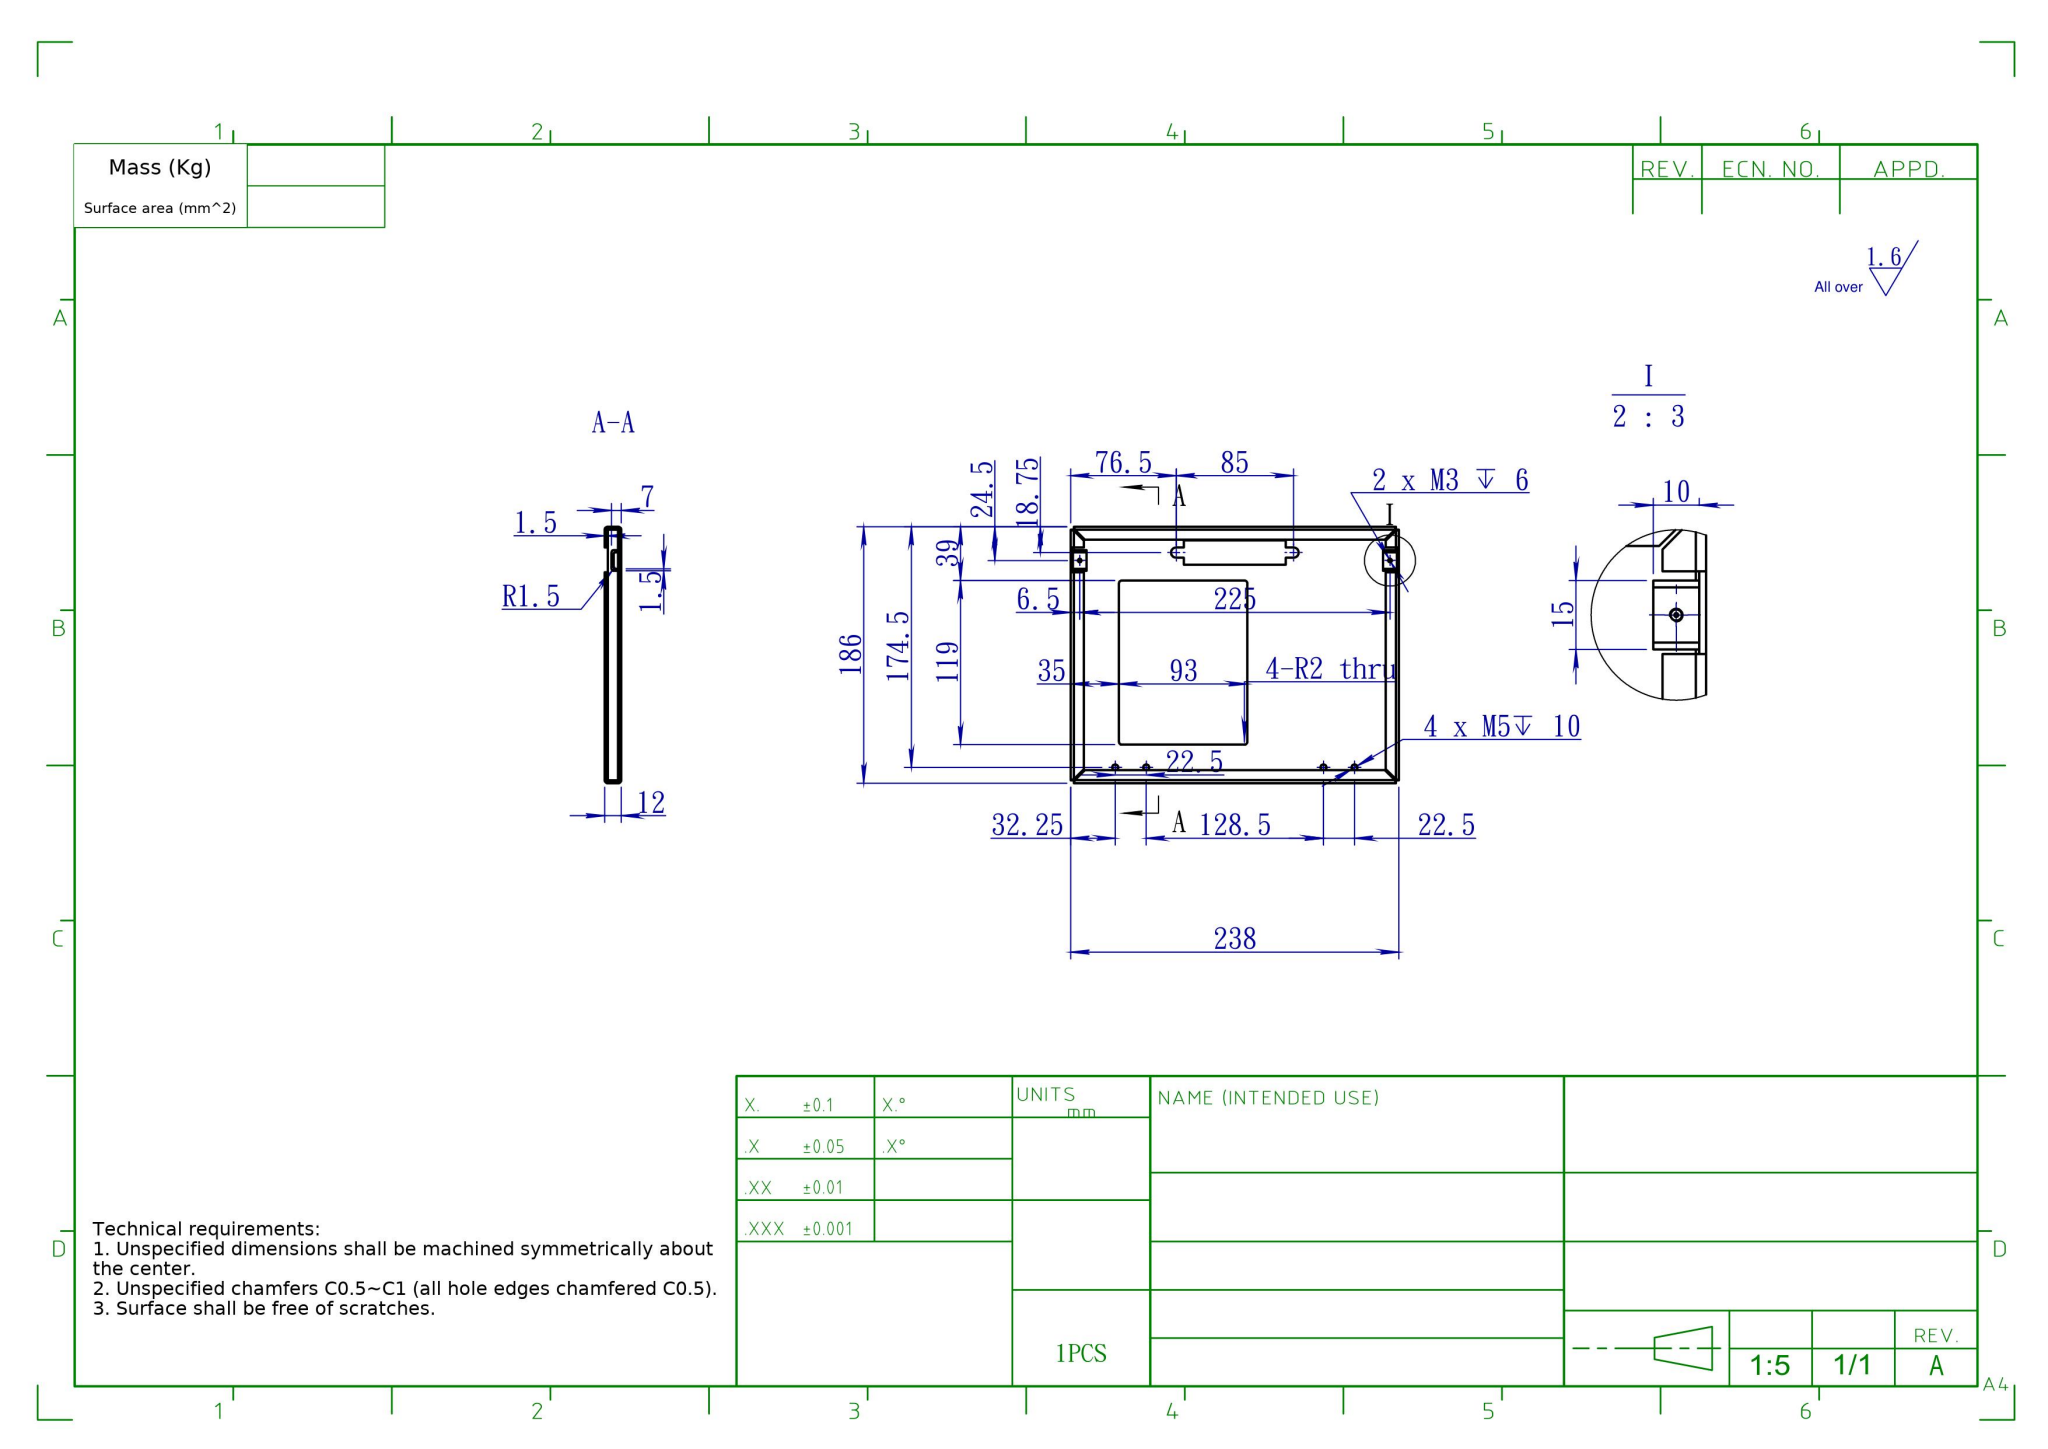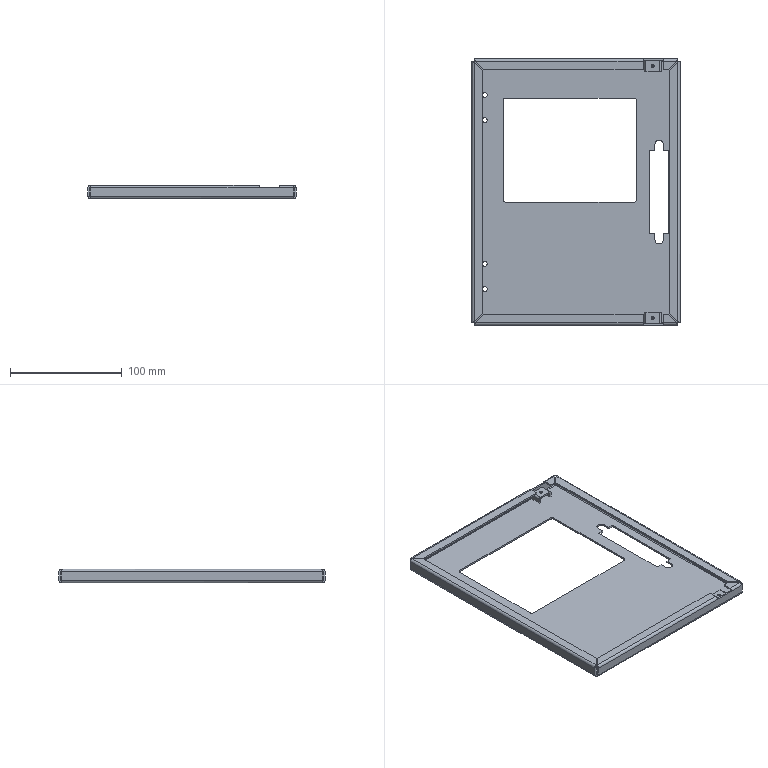Part | SolidWorks | mm | 1 solid | 154 faces | box 186 x 238 x 12 mm | volume 68779 mm3 | plane 84 | cylinder 50 | spline 16 | cone 4 | commonest cylinder face diameters 1.473 x14 4.473 x10 4.2 x8 3 x8 2.5 x4 4 x4 7.5 x2